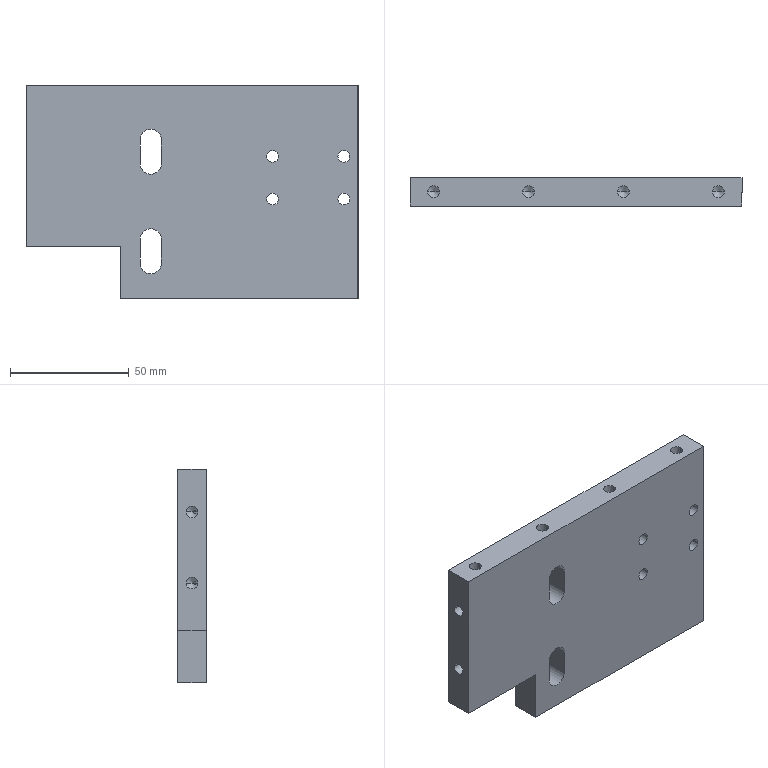Component | SolidWorks | 17081801-804-011A-1 | 1 solid | 72 faces | box 140 x 12 x 90 mm | volume 132790 mm3 | cylinder 36 | cone 24 | plane 12 | commonest cylinder face diameters 5 x32 9 x4 | material Q235
build123d program:
from build123d import *

# Parameters (mm, degrees)
SKETCH1_W                     = 12
SKETCH1_H                     = 90
BOSS_EXTRUDE1_DEPTH           = 40
SKETCH5_W                     = 12
SKETCH5_H                     = 68
BOSS_EXTRUDE3_DEPTH           = 60
M6_TAPPED_HOLE1_D             = 5
M6_TAPPED_HOLE1_DEPTH         = 13
M6_TAPPED_HOLE1_TIP           = 1.502
M6_TAPPED_HOLE2_D             = 5
M6_TAPPED_HOLE2_DEPTH         = 13
M6_TAPPED_HOLE2_TIP           = 1.502
M6_TAPPED_HOLE3_D             = 5
M6_TAPPED_HOLE3_DEPTH         = 15
M6_TAPPED_HOLE3_TIP           = 1.502
SKETCH12_W                    = 12
SKETCH12_H                    = 22
BOSS_EXTRUDE4_DEPTH           = 20
CUT_EXTRUDE2_DEPTH            = 136.07
M6_TAPPED_HOLE4_D             = 5
M6_TAPPED_HOLE4_DEPTH         = 15
M6_TAPPED_HOLE4_TIP           = 1.502
SIZE_MM_DOWEL_PIN_HOLE1_D     = 5
SIZE_MM_DOWEL_PIN_HOLE1_DEPTH = 10
SIZE_MM_DOWEL_PIN_HOLE1_TIP   = 1.502


with BuildPart() as part:
    # Sketch1 → Boss-Extrude1 (new, symmetric)
    with BuildSketch(Plane.XY):
        with Locations((0, 45)):
            Rectangle(SKETCH1_W, SKETCH1_H)
    extrude(amount=BOSS_EXTRUDE1_DEPTH, both=True)

    # Sketch5 → Boss-Extrude3 (add)
    with BuildSketch(Plane.XY.offset(40)):
        with Locations((0, 56)):
            Rectangle(SKETCH5_W, SKETCH5_H)
    extrude(amount=BOSS_EXTRUDE3_DEPTH)

    # M6 Tapped Hole1
    with Locations(Plane(origin=(0, 90, 0), x_dir=(1, 0, 0), z_dir=(0, 1, 0))):
        with Locations((0, 30), (0, -10), (0, -50), (0, -90)):
            Hole(M6_TAPPED_HOLE1_D / 2, depth=M6_TAPPED_HOLE1_DEPTH)
            with Locations((0, 0, -(M6_TAPPED_HOLE1_DEPTH + M6_TAPPED_HOLE1_TIP / 2))):  # 118° drill point
                Cone(0, M6_TAPPED_HOLE1_D / 2, M6_TAPPED_HOLE1_TIP, mode=Mode.SUBTRACT)

    # M6 Tapped Hole2
    with Locations(Plane.XY.offset(100)):
        with Locations((0, 72), (0, 42)):
            Hole(M6_TAPPED_HOLE2_D / 2, depth=M6_TAPPED_HOLE2_DEPTH)
            with Locations((0, 0, -(M6_TAPPED_HOLE2_DEPTH + M6_TAPPED_HOLE2_TIP / 2))):  # 118° drill point
                Cone(0, M6_TAPPED_HOLE2_D / 2, M6_TAPPED_HOLE2_TIP, mode=Mode.SUBTRACT)

    # M6 Tapped Hole3
    with Locations(Plane(origin=(6, 0, 0), x_dir=(0, 0, -1), z_dir=(1, 0, 0))):
        with Locations((34, 60), (34, 42), (4, 42), (4, 60)):
            Hole(M6_TAPPED_HOLE3_D / 2, depth=M6_TAPPED_HOLE3_DEPTH)
            with Locations((0, 0, -(M6_TAPPED_HOLE3_DEPTH + M6_TAPPED_HOLE3_TIP / 2))):  # 118° drill point
                Cone(0, M6_TAPPED_HOLE3_D / 2, M6_TAPPED_HOLE3_TIP, mode=Mode.SUBTRACT)

    # Sketch12 → Boss-Extrude4 (add)
    with BuildSketch(Plane.XY.offset(40)):
        with Locations((0, 11)):
            Rectangle(SKETCH12_W, SKETCH12_H)
    extrude(amount=BOSS_EXTRUDE4_DEPTH)

    # Sketch14 → Cut-Extrude2 (cut, through all)
    with BuildSketch(Plane(origin=(6, 0, 0), x_dir=(0, 0, -1), z_dir=(1, 0, 0))):
        with BuildLine():
            Line((-42.9, 67), (-42.9, 57))
            ThreePointArc((-42.9, 57), (-47.4, 52.5), (-51.9, 57))
            Line((-51.9, 57), (-51.9, 67))
            ThreePointArc((-51.9, 67), (-47.4, 71.5), (-42.9, 67))
        make_face()
        with BuildLine():
            Line((-42.9, 25), (-42.9, 15))
            ThreePointArc((-42.9, 15), (-47.4, 10.5), (-51.9, 15))
            Line((-51.9, 15), (-51.9, 25))
            ThreePointArc((-51.9, 25), (-47.4, 29.5), (-42.9, 25))
        make_face()
    extrude(amount=-CUT_EXTRUDE2_DEPTH, mode=Mode.SUBTRACT)

    # M6 Tapped Hole4
    with Locations(Plane(origin=(0, 0, 0), x_dir=(-1, 0, 0), z_dir=(0, -1, 0))):
        with Locations((0, 15), (0, 35), (0, -15), (0, -35)):
            Hole(M6_TAPPED_HOLE4_D / 2, depth=M6_TAPPED_HOLE4_DEPTH)
            with Locations((0, 0, -(M6_TAPPED_HOLE4_DEPTH + M6_TAPPED_HOLE4_TIP / 2))):  # 118° drill point
                Cone(0, M6_TAPPED_HOLE4_D / 2, M6_TAPPED_HOLE4_TIP, mode=Mode.SUBTRACT)

    # Size mm Dowel Pin Hole1
    with Locations(Plane(origin=(0, 0, 0), x_dir=(-1, 0, 0), z_dir=(0, -1, 0))):
        with Locations((0, 25), (0, -25)):
            Hole(SIZE_MM_DOWEL_PIN_HOLE1_D / 2, depth=SIZE_MM_DOWEL_PIN_HOLE1_DEPTH)
            with Locations((0, 0, -(SIZE_MM_DOWEL_PIN_HOLE1_DEPTH + SIZE_MM_DOWEL_PIN_HOLE1_TIP / 2))):  # 118° drill point
                Cone(0, SIZE_MM_DOWEL_PIN_HOLE1_D / 2, SIZE_MM_DOWEL_PIN_HOLE1_TIP, mode=Mode.SUBTRACT)


solid = part.part

# Placed as in the assembly
solid = solid.moved(Location((-14.5, 1974.4, 132), (90, -90, 0)))